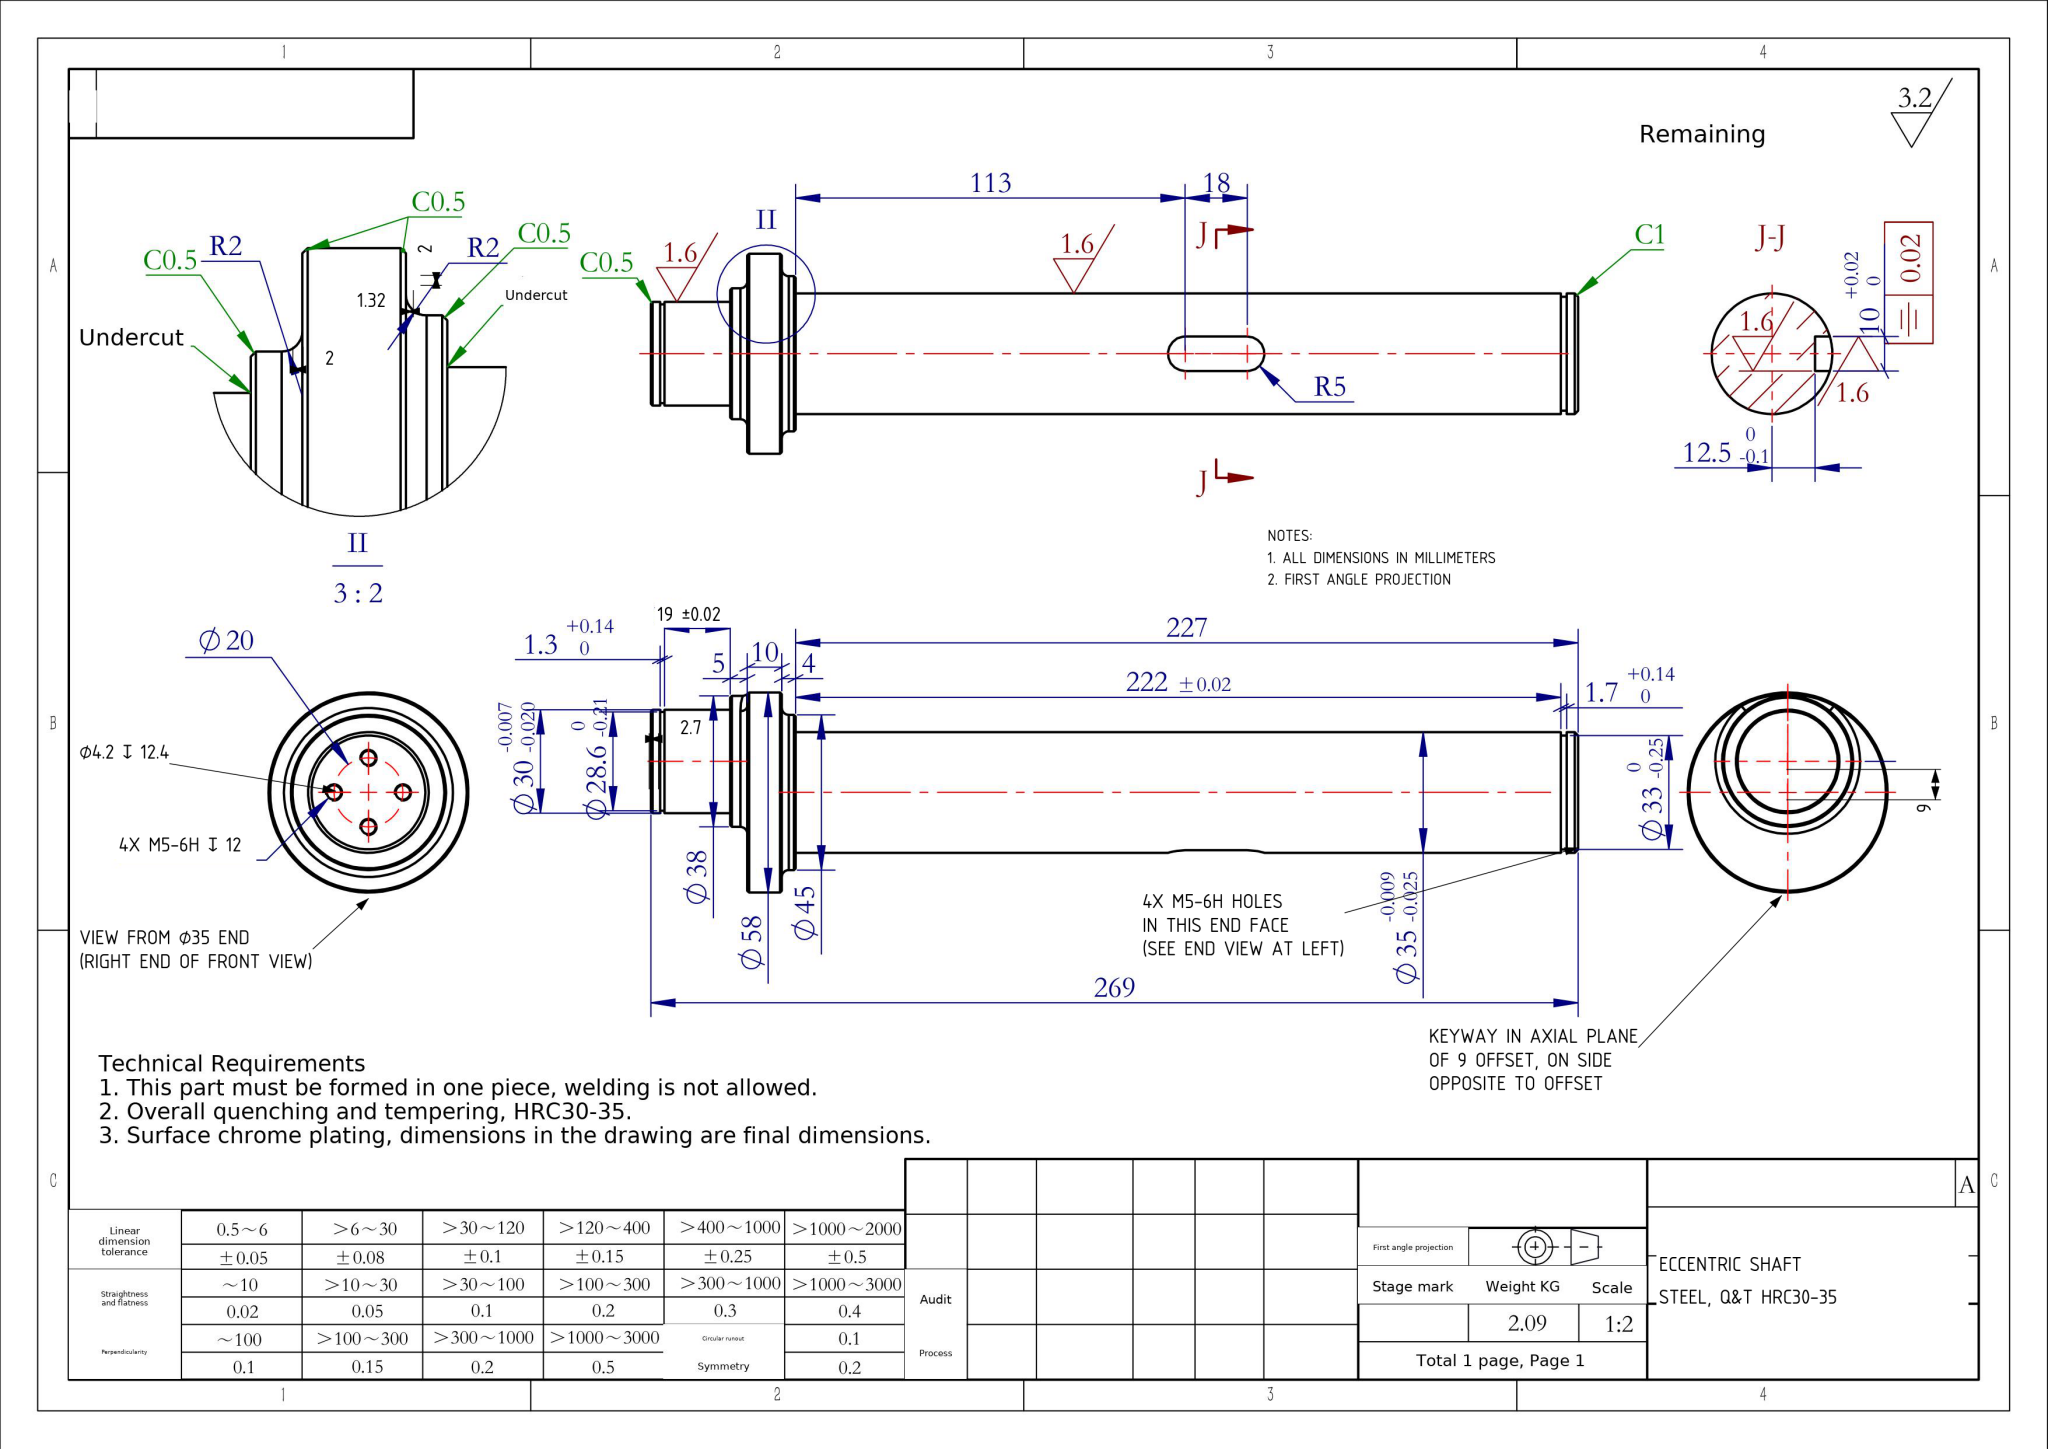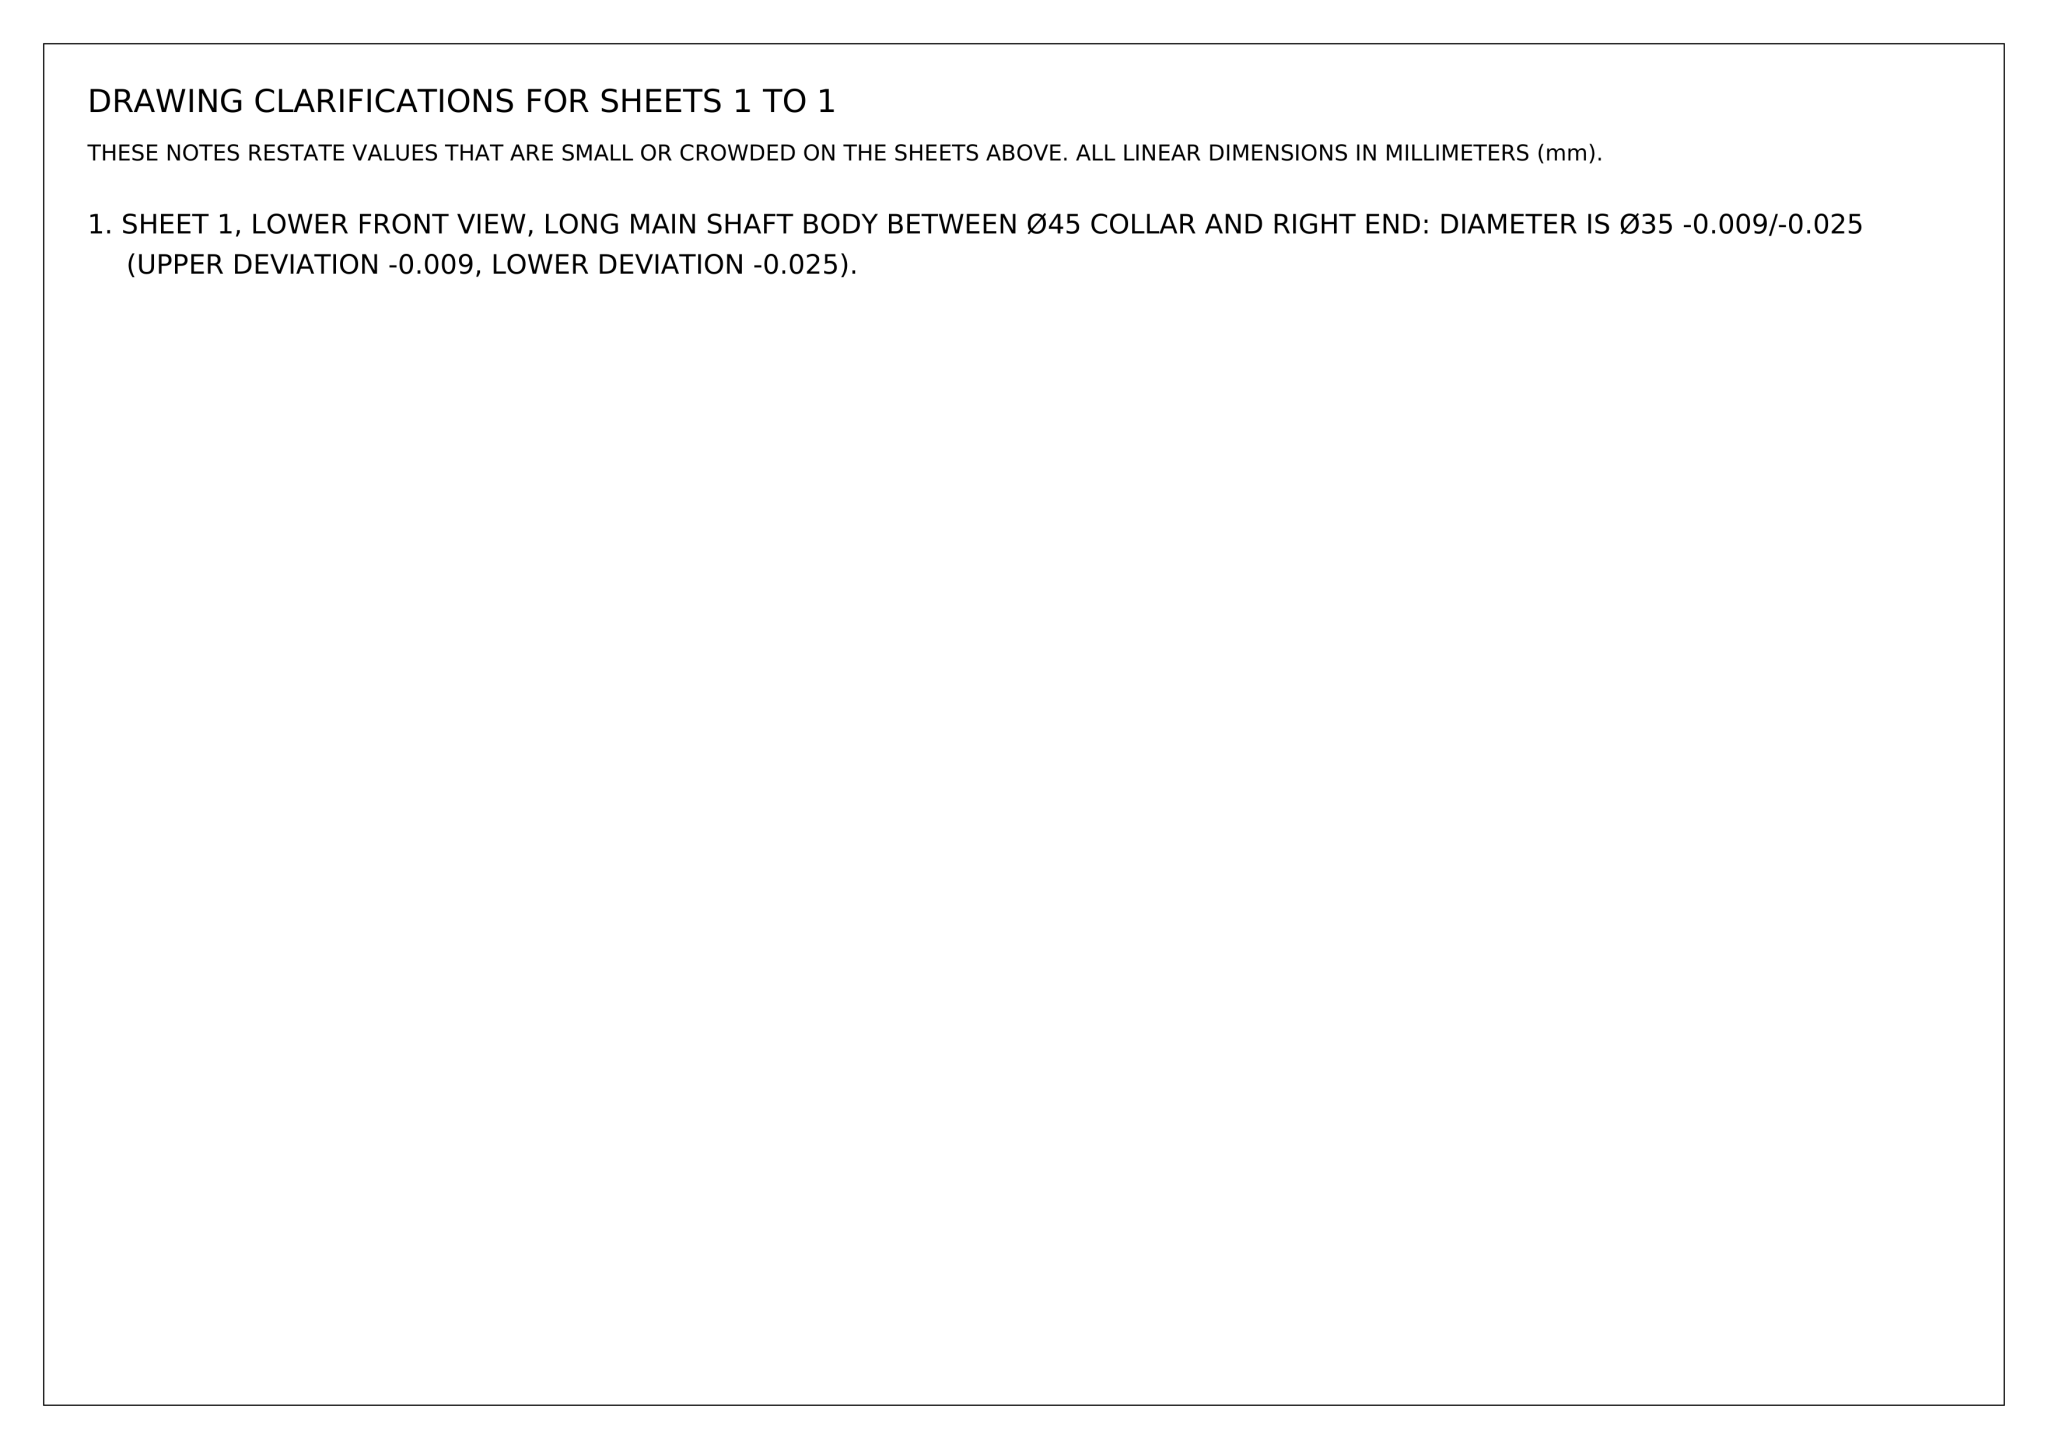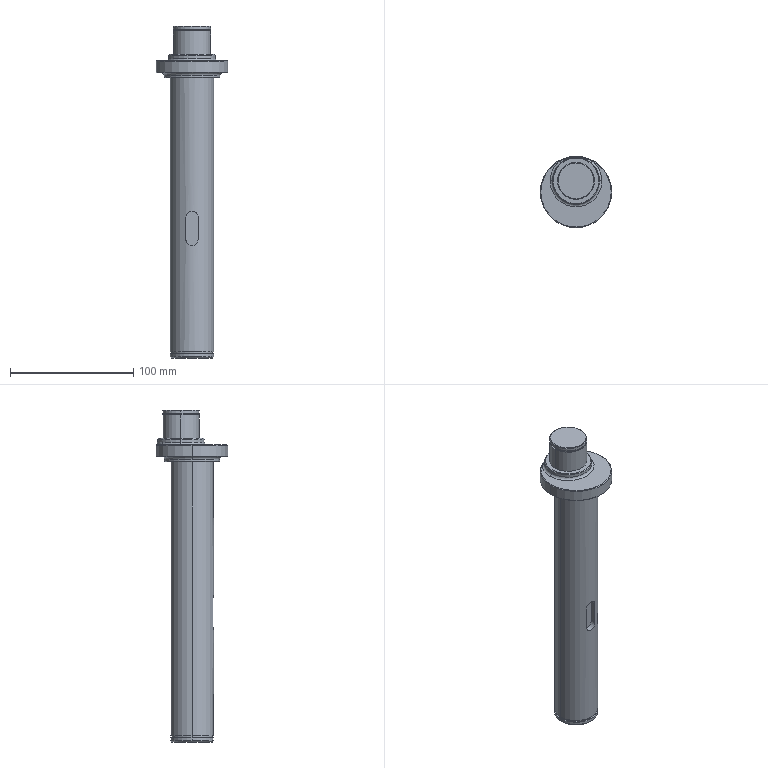Part | NX | mm | 1 solid | 68 faces | box 58 x 58 x 269 mm | volume 270975 mm3 | cylinder 29 | cone 20 | plane 13 | torus 5 | spline 1 | commonest cylinder face diameters 4.2 x8 35 x4 30 x4 10 x3 33 x2 28.6 x2 38 x2 45 x2